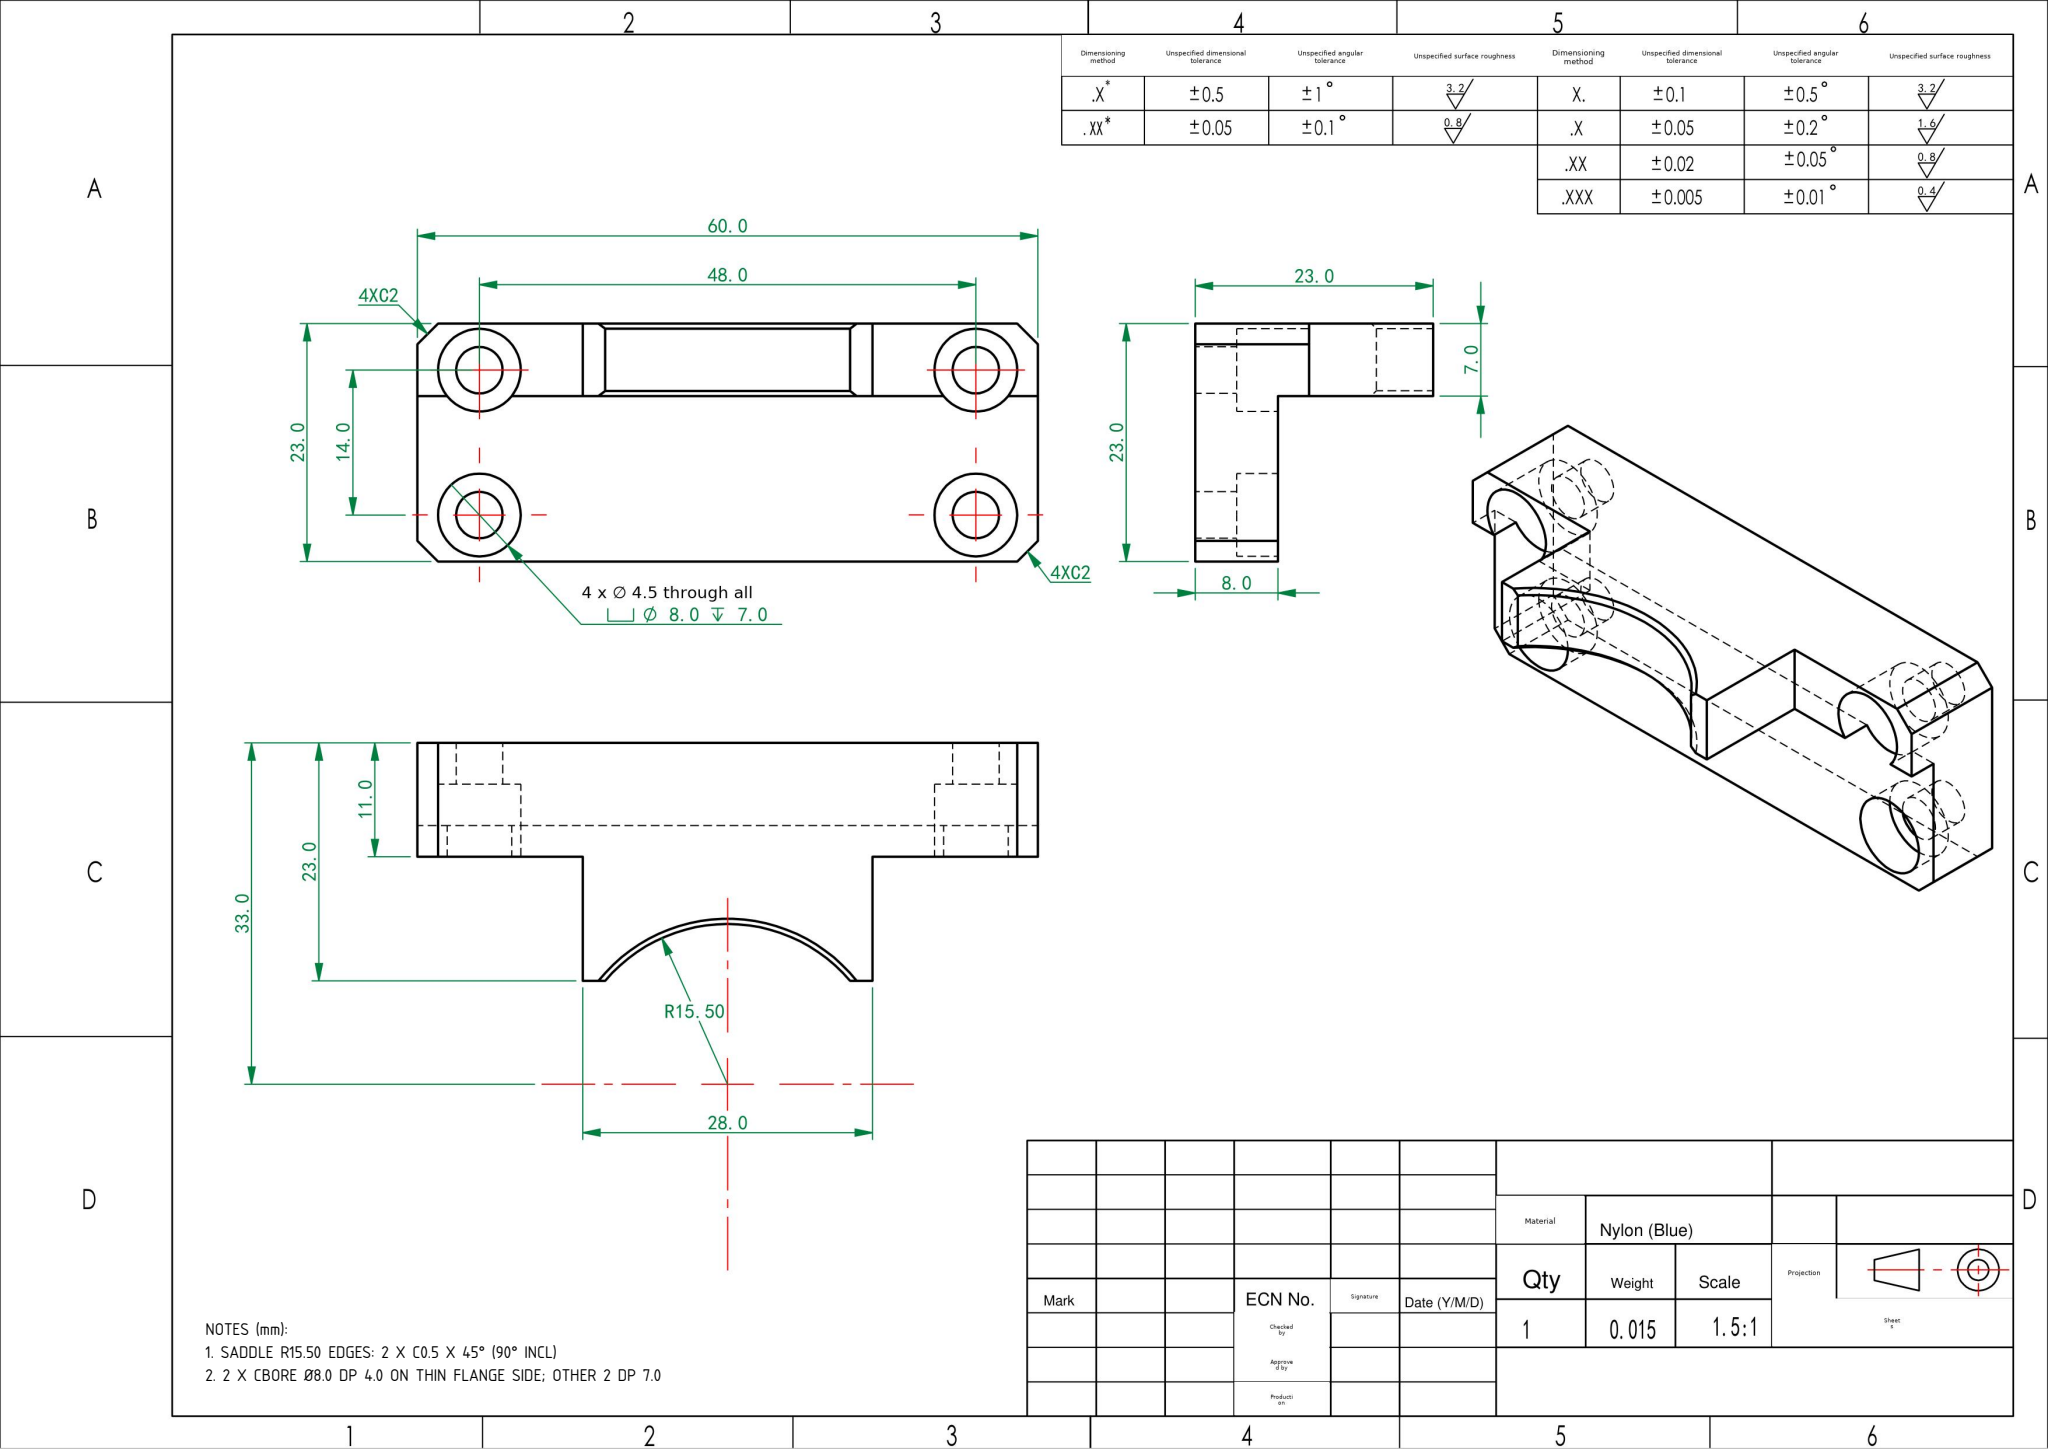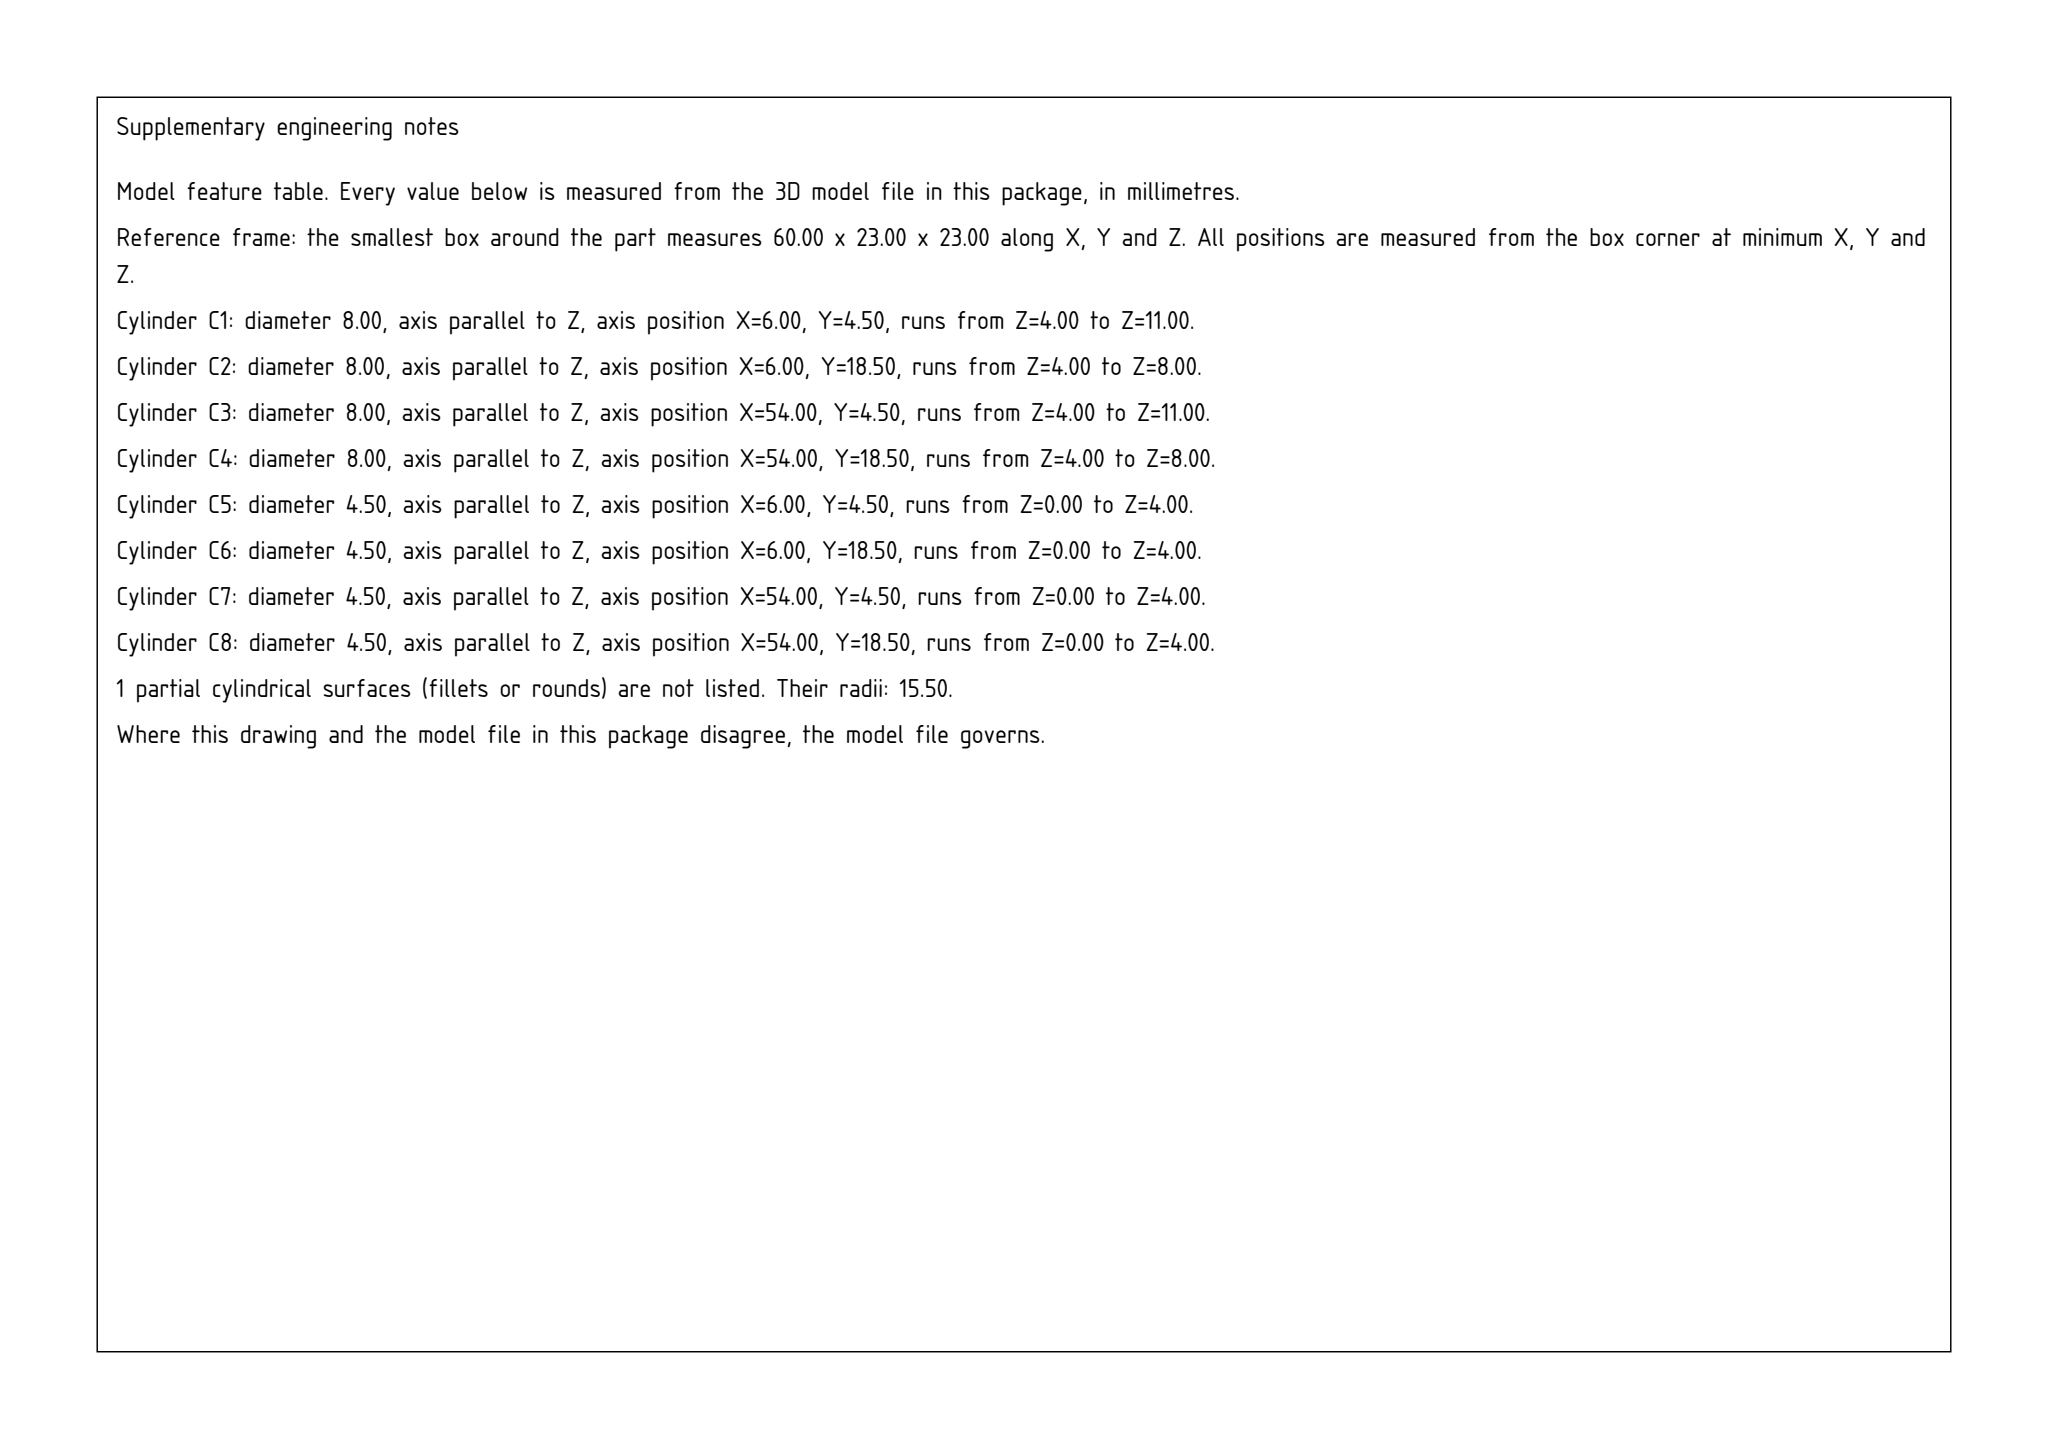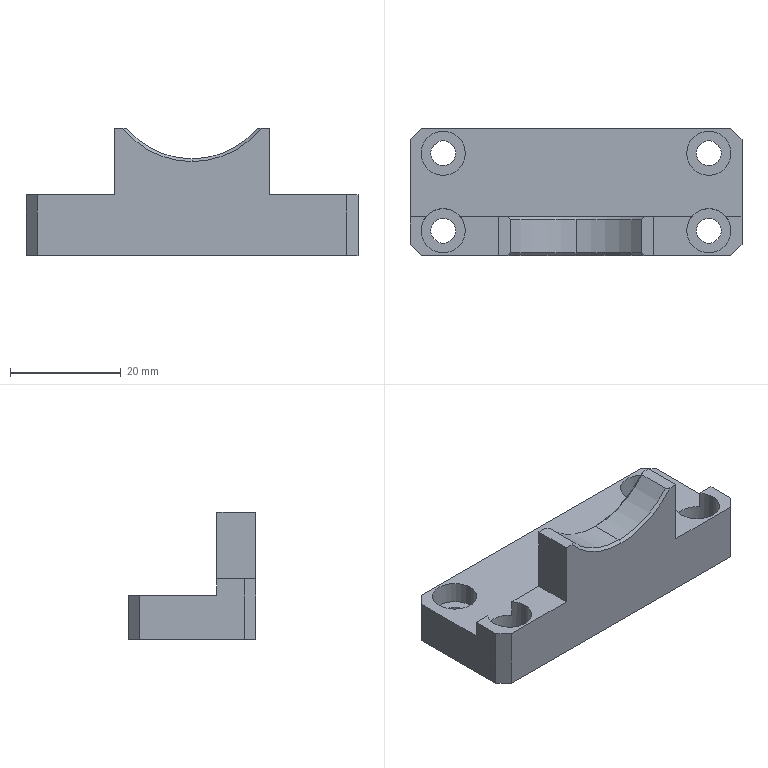Part | SolidWorks | mm | 1 solid | 44 faces | box 60 x 23 x 23 mm | volume 12615 mm3 | plane 23 | cylinder 18 | cone 3 | commonest cylinder face diameters 4.5 x8 8 x8 31 x2
Drawing notes:
SADDLE R15.50 EDGES: 2 X C0.5 X 45° (90° INCL) | from the solid: cones 90° incl, ref dia 31.0 (2 off) vs saddle cyl dia 31.0; outer ref dia 32.0 gives 0.5 radial leg
2 X CBORE Ø8.0 DP 4.0 ON THIN FLANGE SIDE; OTHER 2 DP 7.0 | from the solid: Ø8 z-cyls at y=18.5 length 4.0 (x=6,54); Ø8 z-cyls at y=4.5 length 7.0 (x=6,54)
build123d program:
from build123d import *

# Parameters (mm, degrees)
SKETCH1_W                                          = 60
SKETCH1_H                                          = 23
BOSS_EXTRUDE1_DEPTH                                = 23
SKETCH4_W                                          = 60
SKETCH4_H                                          = 16
CUT_EXTRUDE1_DEPTH                                 = 15
SKETCH7_R                                          = 15.5
CUT_EXTRUDE2_DEPTH                                 = 31
SKETCH8_OUTSIDE_W                                  = 75.65
SKETCH8_OUTSIDE_H                                  = 38.65
SKETCH8_OUTSIDE_W_2                                = 28
SKETCH8_OUTSIDE_H_2                                = 23
CUT_EXTRUDE3_DEPTH                                 = 12
HOLE_SIZE_ACCORDING_TO_HEX_SOCKET_HEAD_D           = 4.5
HOLE_SIZE_ACCORDING_TO_HEX_SOCKET_HEAD_CBORE_D     = 8
HOLE_SIZE_ACCORDING_TO_HEX_SOCKET_HEAD_CBORE_DEPTH = 7
CHAMFER1_SIZE                                      = 2
CHAMFER2_SIZE                                      = 0.5


with BuildPart() as part:
    # Sketch1 → Boss-Extrude1 (new body)
    with BuildSketch(Plane.XY):
        Rectangle(SKETCH1_W, SKETCH1_H)
    extrude(amount=BOSS_EXTRUDE1_DEPTH)

    # Sketch4 → Cut-Extrude1 (cut)
    with BuildSketch(Plane.XY.offset(23)):
        with Locations((0, 3.5)):
            Rectangle(SKETCH4_W, SKETCH4_H)
    extrude(amount=-CUT_EXTRUDE1_DEPTH, mode=Mode.SUBTRACT)

    # Sketch7 → Cut-Extrude2 (cut)
    with BuildSketch(Plane.XZ.offset(11.5)):
        with Locations((0, 33)):
            Circle(SKETCH7_R)
    extrude(amount=-CUT_EXTRUDE2_DEPTH, mode=Mode.SUBTRACT)

    # Sketch8 outside → Cut-Extrude3 (cut)
    with BuildSketch(Plane.XY.offset(23)):
        Rectangle(SKETCH8_OUTSIDE_W, SKETCH8_OUTSIDE_H)
        Rectangle(SKETCH8_OUTSIDE_W_2, SKETCH8_OUTSIDE_H_2, mode=Mode.SUBTRACT)
    extrude(amount=-CUT_EXTRUDE3_DEPTH, mode=Mode.SUBTRACT)

    # Hole Size _According to_ Hex Socket Head (through all)
    with Locations(Plane(origin=(-24, 7, 11), x_dir=(1, 0, 0), z_dir=(0, 0, 1))):
        with Locations((0, 0), (0, -14), (48, -14), (48, 0)):
            CounterBoreHole(HOLE_SIZE_ACCORDING_TO_HEX_SOCKET_HEAD_D / 2, HOLE_SIZE_ACCORDING_TO_HEX_SOCKET_HEAD_CBORE_D / 2, HOLE_SIZE_ACCORDING_TO_HEX_SOCKET_HEAD_CBORE_DEPTH)

    # Chamfer1
    chamfer1_edges = [part.edges().sort_by_distance(p)[0] for p in [
        (-30, 11.5, 4),
        (30, 11.5, 4),
        (-30, -11.5, 5.5),
        (30, -11.5, 5.5),
    ]]
    chamfer(chamfer1_edges, length=CHAMFER1_SIZE)

    # Chamfer2
    chamfer2_edges = [part.edges().sort_by_distance(p)[0] for p in [
        (0, -4.5, 17.5),
        (0, -11.5, 17.5),
    ]]
    chamfer(chamfer2_edges, length=CHAMFER2_SIZE)


solid = part.part